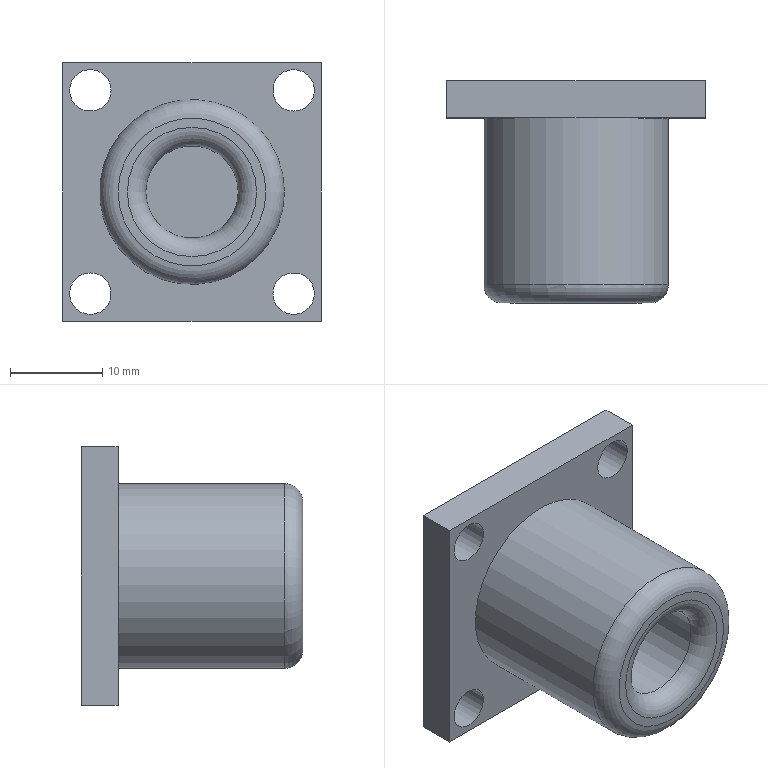Component | NX | INTERFACE_2 | 1 solid | 16 faces | box 28 x 24 x 28 mm | volume 7513 mm3 | plane 8 | cylinder 6 | torus 2 | commonest cylinder face diameters 4.5 x4 20 x1 10 x1
STEP:
#1=CARTESIAN_POINT('',(0.,0.,0.));
#2=DIRECTION('',(0.,0.,1.));
#3=DIRECTION('',(1.,0.,0.));
#4=AXIS2_PLACEMENT_3D('',#1,#2,#3);
#5=CARTESIAN_POINT('',(-14.,-309.,-187.));
#6=VERTEX_POINT('',#5);
#7=CARTESIAN_POINT('',(-14.,-309.,-215.));
#8=VERTEX_POINT('',#7);
#9=CARTESIAN_POINT('',(-14.,-309.,-187.));
#10=DIRECTION('',(0.,0.,-1.));
#11=VECTOR('',#10,1.);
#12=LINE('',#9,#11);
#13=CARTESIAN_POINT('',(-14.,-305.,-187.));
#14=DIRECTION('',(-1.,0.,0.));
#15=DIRECTION('',(0.,-1.,0.));
#16=AXIS2_PLACEMENT_3D('',#13,#14,#15);
#17=PLANE('',#16);
#18=CARTESIAN_POINT('',(4.,0.));
#19=DIRECTION('',(0.,-1.));
#20=VECTOR('',#19,1.);
#21=LINE('',#18,#20);
#22=(GEOMETRIC_REPRESENTATION_CONTEXT(2)PARAMETRIC_REPRESENTATION_CONTEXT()REPRESENTATION_CONTEXT('',''));
#23=DEFINITIONAL_REPRESENTATION('',(#21),#22);
#24=PCURVE('',#17,#23);
#25=CARTESIAN_POINT('',(-11.,-309.,-212.));
#26=DIRECTION('',(0.,-1.,0.));
#27=DIRECTION('',(1.,0.,0.));
#28=AXIS2_PLACEMENT_3D('',#25,#26,#27);
#29=PLANE('',#28);
#30=CARTESIAN_POINT('',(-3.,25.));
#31=DIRECTION('',(0.,-1.));
#32=VECTOR('',#31,1.);
#33=LINE('',#30,#32);
#34=(GEOMETRIC_REPRESENTATION_CONTEXT(2)PARAMETRIC_REPRESENTATION_CONTEXT()REPRESENTATION_CONTEXT('',''));
#35=DEFINITIONAL_REPRESENTATION('',(#33),#34);
#36=PCURVE('',#29,#35);
#37=SURFACE_CURVE('',#12,(#24,#36),.PCURVE_S1.);
#38=EDGE_CURVE('',#6,#8,#37,.T.);
#39=ORIENTED_EDGE('',*,*,#38,.F.);
#40=CARTESIAN_POINT('',(-14.,-305.,-187.));
#41=VERTEX_POINT('',#40);
#42=CARTESIAN_POINT('',(-14.,-305.,-187.));
#43=DIRECTION('',(0.,-1.,0.));
#44=VECTOR('',#43,1.);
#45=LINE('',#42,#44);
#46=CARTESIAN_POINT('',(0.,0.));
#47=DIRECTION('',(1.,0.));
#48=VECTOR('',#47,1.);
#49=LINE('',#46,#48);
#50=(GEOMETRIC_REPRESENTATION_CONTEXT(2)PARAMETRIC_REPRESENTATION_CONTEXT()REPRESENTATION_CONTEXT('',''));
#51=DEFINITIONAL_REPRESENTATION('',(#49),#50);
#52=PCURVE('',#17,#51);
#53=CARTESIAN_POINT('',(14.,-305.,-187.));
#54=DIRECTION('',(0.,0.,1.));
#55=DIRECTION('',(0.,-1.,0.));
#56=AXIS2_PLACEMENT_3D('',#53,#54,#55);
#57=PLANE('',#56);
#58=CARTESIAN_POINT('',(0.,-28.));
#59=DIRECTION('',(1.,0.));
#60=VECTOR('',#59,1.);
#61=LINE('',#58,#60);
#62=(GEOMETRIC_REPRESENTATION_CONTEXT(2)PARAMETRIC_REPRESENTATION_CONTEXT()REPRESENTATION_CONTEXT('',''));
#63=DEFINITIONAL_REPRESENTATION('',(#61),#62);
#64=PCURVE('',#57,#63);
#65=SURFACE_CURVE('',#45,(#52,#64),.PCURVE_S1.);
#66=EDGE_CURVE('',#41,#6,#65,.T.);
#67=ORIENTED_EDGE('',*,*,#66,.F.);
#68=CARTESIAN_POINT('',(-14.,-305.,-215.));
#69=VERTEX_POINT('',#68);
#70=CARTESIAN_POINT('',(-14.,-305.,-187.));
#71=DIRECTION('',(0.,0.,-1.));
#72=VECTOR('',#71,1.);
#73=LINE('',#70,#72);
#74=CARTESIAN_POINT('',(0.,0.));
#75=DIRECTION('',(0.,-1.));
#76=VECTOR('',#75,1.);
#77=LINE('',#74,#76);
#78=(GEOMETRIC_REPRESENTATION_CONTEXT(2)PARAMETRIC_REPRESENTATION_CONTEXT()REPRESENTATION_CONTEXT('',''));
#79=DEFINITIONAL_REPRESENTATION('',(#77),#78);
#80=PCURVE('',#17,#79);
#81=CARTESIAN_POINT('',(-11.,-305.,-212.));
#82=DIRECTION('',(0.,-1.,0.));
#83=DIRECTION('',(1.,0.,0.));
#84=AXIS2_PLACEMENT_3D('',#81,#82,#83);
#85=PLANE('',#84);
#86=CARTESIAN_POINT('',(-3.,25.));
#87=DIRECTION('',(0.,-1.));
#88=VECTOR('',#87,1.);
#89=LINE('',#86,#88);
#90=(GEOMETRIC_REPRESENTATION_CONTEXT(2)PARAMETRIC_REPRESENTATION_CONTEXT()REPRESENTATION_CONTEXT('',''));
#91=DEFINITIONAL_REPRESENTATION('',(#89),#90);
#92=PCURVE('',#85,#91);
#93=SURFACE_CURVE('',#73,(#80,#92),.PCURVE_S1.);
#94=EDGE_CURVE('',#41,#69,#93,.T.);
#95=ORIENTED_EDGE('',*,*,#94,.T.);
#96=CARTESIAN_POINT('',(-14.,-305.,-215.));
#97=DIRECTION('',(0.,-1.,0.));
#98=VECTOR('',#97,1.);
#99=LINE('',#96,#98);
#100=CARTESIAN_POINT('',(0.,-28.));
#101=DIRECTION('',(1.,0.));
#102=VECTOR('',#101,1.);
#103=LINE('',#100,#102);
#104=(GEOMETRIC_REPRESENTATION_CONTEXT(2)PARAMETRIC_REPRESENTATION_CONTEXT()REPRESENTATION_CONTEXT('',''));
#105=DEFINITIONAL_REPRESENTATION('',(#103),#104);
#106=PCURVE('',#17,#105);
#107=CARTESIAN_POINT('',(-14.,-305.,-215.));
#108=DIRECTION('',(0.,0.,-1.));
#109=DIRECTION('',(0.,1.,0.));
#110=AXIS2_PLACEMENT_3D('',#107,#108,#109);
#111=PLANE('',#110);
#112=CARTESIAN_POINT('',(0.,0.));
#113=DIRECTION('',(-1.,0.));
#114=VECTOR('',#113,1.);
#115=LINE('',#112,#114);
#116=(GEOMETRIC_REPRESENTATION_CONTEXT(2)PARAMETRIC_REPRESENTATION_CONTEXT()REPRESENTATION_CONTEXT('',''));
#117=DEFINITIONAL_REPRESENTATION('',(#115),#116);
#118=PCURVE('',#111,#117);
#119=SURFACE_CURVE('',#99,(#106,#118),.PCURVE_S1.);
#120=EDGE_CURVE('',#69,#8,#119,.T.);
#121=ORIENTED_EDGE('',*,*,#120,.T.);
#122=EDGE_LOOP('',(#39,#67,#95,#121));
#123=FACE_BOUND('',#122,.T.);
#124=ADVANCED_FACE('',(#123),#17,.T.);
#125=CARTESIAN_POINT('',(14.,-309.,-215.));
#126=VERTEX_POINT('',#125);
#127=CARTESIAN_POINT('',(-14.,-309.,-215.));
#128=DIRECTION('',(1.,0.,0.));
#129=VECTOR('',#128,1.);
#130=LINE('',#127,#129);
#131=CARTESIAN_POINT('',(-4.,0.));
#132=DIRECTION('',(0.,1.));
#133=VECTOR('',#132,1.);
#134=LINE('',#131,#133);
#135=(GEOMETRIC_REPRESENTATION_CONTEXT(2)PARAMETRIC_REPRESENTATION_CONTEXT()REPRESENTATION_CONTEXT('',''));
#136=DEFINITIONAL_REPRESENTATION('',(#134),#135);
#137=PCURVE('',#111,#136);
#138=CARTESIAN_POINT('',(-3.,-3.));
#139=DIRECTION('',(1.,0.));
#140=VECTOR('',#139,1.);
#141=LINE('',#138,#140);
#142=(GEOMETRIC_REPRESENTATION_CONTEXT(2)PARAMETRIC_REPRESENTATION_CONTEXT()REPRESENTATION_CONTEXT('',''));
#143=DEFINITIONAL_REPRESENTATION('',(#141),#142);
#144=PCURVE('',#29,#143);
#145=SURFACE_CURVE('',#130,(#137,#144),.PCURVE_S1.);
#146=EDGE_CURVE('',#8,#126,#145,.T.);
#147=ORIENTED_EDGE('',*,*,#146,.F.);
#148=ORIENTED_EDGE('',*,*,#120,.F.);
#149=CARTESIAN_POINT('',(14.,-305.,-215.));
#150=VERTEX_POINT('',#149);
#151=CARTESIAN_POINT('',(-14.,-305.,-215.));
#152=DIRECTION('',(1.,0.,0.));
#153=VECTOR('',#152,1.);
#154=LINE('',#151,#153);
#155=CARTESIAN_POINT('',(0.,0.));
#156=DIRECTION('',(0.,1.));
#157=VECTOR('',#156,1.);
#158=LINE('',#155,#157);
#159=(GEOMETRIC_REPRESENTATION_CONTEXT(2)PARAMETRIC_REPRESENTATION_CONTEXT()REPRESENTATION_CONTEXT('',''));
#160=DEFINITIONAL_REPRESENTATION('',(#158),#159);
#161=PCURVE('',#111,#160);
#162=CARTESIAN_POINT('',(-3.,-3.));
#163=DIRECTION('',(1.,0.));
#164=VECTOR('',#163,1.);
#165=LINE('',#162,#164);
#166=(GEOMETRIC_REPRESENTATION_CONTEXT(2)PARAMETRIC_REPRESENTATION_CONTEXT()REPRESENTATION_CONTEXT('',''));
#167=DEFINITIONAL_REPRESENTATION('',(#165),#166);
#168=PCURVE('',#85,#167);
#169=SURFACE_CURVE('',#154,(#161,#168),.PCURVE_S1.);
#170=EDGE_CURVE('',#69,#150,#169,.T.);
#171=ORIENTED_EDGE('',*,*,#170,.T.);
#172=CARTESIAN_POINT('',(14.,-305.,-215.));
#173=DIRECTION('',(0.,-1.,0.));
#174=VECTOR('',#173,1.);
#175=LINE('',#172,#174);
#176=CARTESIAN_POINT('',(0.,28.));
#177=DIRECTION('',(-1.,0.));
#178=VECTOR('',#177,1.);
#179=LINE('',#176,#178);
#180=(GEOMETRIC_REPRESENTATION_CONTEXT(2)PARAMETRIC_REPRESENTATION_CONTEXT()REPRESENTATION_CONTEXT('',''));
#181=DEFINITIONAL_REPRESENTATION('',(#179),#180);
#182=PCURVE('',#111,#181);
#183=CARTESIAN_POINT('',(14.,-305.,-215.));
#184=DIRECTION('',(1.,0.,0.));
#185=DIRECTION('',(0.,1.,0.));
#186=AXIS2_PLACEMENT_3D('',#183,#184,#185);
#187=PLANE('',#186);
#188=CARTESIAN_POINT('',(0.,0.));
#189=DIRECTION('',(-1.,0.));
#190=VECTOR('',#189,1.);
#191=LINE('',#188,#190);
#192=(GEOMETRIC_REPRESENTATION_CONTEXT(2)PARAMETRIC_REPRESENTATION_CONTEXT()REPRESENTATION_CONTEXT('',''));
#193=DEFINITIONAL_REPRESENTATION('',(#191),#192);
#194=PCURVE('',#187,#193);
#195=SURFACE_CURVE('',#175,(#182,#194),.PCURVE_S1.);
#196=EDGE_CURVE('',#150,#126,#195,.T.);
#197=ORIENTED_EDGE('',*,*,#196,.T.);
#198=EDGE_LOOP('',(#147,#148,#171,#197));
#199=FACE_BOUND('',#198,.T.);
#200=ADVANCED_FACE('',(#199),#111,.T.);
#201=CARTESIAN_POINT('',(14.,-309.,-187.));
#202=VERTEX_POINT('',#201);
#203=CARTESIAN_POINT('',(14.,-309.,-215.));
#204=DIRECTION('',(0.,0.,1.));
#205=VECTOR('',#204,1.);
#206=LINE('',#203,#205);
#207=CARTESIAN_POINT('',(-4.,0.));
#208=DIRECTION('',(0.,1.));
#209=VECTOR('',#208,1.);
#210=LINE('',#207,#209);
#211=(GEOMETRIC_REPRESENTATION_CONTEXT(2)PARAMETRIC_REPRESENTATION_CONTEXT()REPRESENTATION_CONTEXT('',''));
#212=DEFINITIONAL_REPRESENTATION('',(#210),#211);
#213=PCURVE('',#187,#212);
#214=CARTESIAN_POINT('',(25.,-3.));
#215=DIRECTION('',(0.,1.));
#216=VECTOR('',#215,1.);
#217=LINE('',#214,#216);
#218=(GEOMETRIC_REPRESENTATION_CONTEXT(2)PARAMETRIC_REPRESENTATION_CONTEXT()REPRESENTATION_CONTEXT('',''));
#219=DEFINITIONAL_REPRESENTATION('',(#217),#218);
#220=PCURVE('',#29,#219);
#221=SURFACE_CURVE('',#206,(#213,#220),.PCURVE_S1.);
#222=EDGE_CURVE('',#126,#202,#221,.T.);
#223=ORIENTED_EDGE('',*,*,#222,.F.);
#224=ORIENTED_EDGE('',*,*,#196,.F.);
#225=CARTESIAN_POINT('',(14.,-305.,-187.));
#226=VERTEX_POINT('',#225);
#227=CARTESIAN_POINT('',(14.,-305.,-215.));
#228=DIRECTION('',(0.,0.,1.));
#229=VECTOR('',#228,1.);
#230=LINE('',#227,#229);
#231=CARTESIAN_POINT('',(0.,0.));
#232=DIRECTION('',(0.,1.));
#233=VECTOR('',#232,1.);
#234=LINE('',#231,#233);
#235=(GEOMETRIC_REPRESENTATION_CONTEXT(2)PARAMETRIC_REPRESENTATION_CONTEXT()REPRESENTATION_CONTEXT('',''));
#236=DEFINITIONAL_REPRESENTATION('',(#234),#235);
#237=PCURVE('',#187,#236);
#238=CARTESIAN_POINT('',(25.,-3.));
#239=DIRECTION('',(0.,1.));
#240=VECTOR('',#239,1.);
#241=LINE('',#238,#240);
#242=(GEOMETRIC_REPRESENTATION_CONTEXT(2)PARAMETRIC_REPRESENTATION_CONTEXT()REPRESENTATION_CONTEXT('',''));
#243=DEFINITIONAL_REPRESENTATION('',(#241),#242);
#244=PCURVE('',#85,#243);
#245=SURFACE_CURVE('',#230,(#237,#244),.PCURVE_S1.);
#246=EDGE_CURVE('',#150,#226,#245,.T.);
#247=ORIENTED_EDGE('',*,*,#246,.T.);
#248=CARTESIAN_POINT('',(14.,-305.,-187.));
#249=DIRECTION('',(0.,-1.,0.));
#250=VECTOR('',#249,1.);
#251=LINE('',#248,#250);
#252=CARTESIAN_POINT('',(0.,28.));
#253=DIRECTION('',(-1.,0.));
#254=VECTOR('',#253,1.);
#255=LINE('',#252,#254);
#256=(GEOMETRIC_REPRESENTATION_CONTEXT(2)PARAMETRIC_REPRESENTATION_CONTEXT()REPRESENTATION_CONTEXT('',''));
#257=DEFINITIONAL_REPRESENTATION('',(#255),#256);
#258=PCURVE('',#187,#257);
#259=CARTESIAN_POINT('',(0.,0.));
#260=DIRECTION('',(1.,0.));
#261=VECTOR('',#260,1.);
#262=LINE('',#259,#261);
#263=(GEOMETRIC_REPRESENTATION_CONTEXT(2)PARAMETRIC_REPRESENTATION_CONTEXT()REPRESENTATION_CONTEXT('',''));
#264=DEFINITIONAL_REPRESENTATION('',(#262),#263);
#265=PCURVE('',#57,#264);
#266=SURFACE_CURVE('',#251,(#258,#265),.PCURVE_S1.);
#267=EDGE_CURVE('',#226,#202,#266,.T.);
#268=ORIENTED_EDGE('',*,*,#267,.T.);
#269=EDGE_LOOP('',(#223,#224,#247,#268));
#270=FACE_BOUND('',#269,.T.);
#271=ADVANCED_FACE('',(#270),#187,.T.);
#272=CARTESIAN_POINT('',(8.75,-305.,-212.));
#273=VERTEX_POINT('',#272);
#274=CARTESIAN_POINT('',(11.,-305.,-212.));
#275=DIRECTION('',(0.,-1.,0.));
#276=DIRECTION('',(-1.,0.,0.));
#277=AXIS2_PLACEMENT_3D('',#274,#275,#276);
#278=CIRCLE('',#277,2.25);
#279=CARTESIAN_POINT('',(11.,-305.,-212.));
#280=DIRECTION('',(0.,-1.,0.));
#281=DIRECTION('',(1.,0.,0.));
#282=AXIS2_PLACEMENT_3D('',#279,#280,#281);
#283=CYLINDRICAL_SURFACE('',#282,2.25);
#284=CARTESIAN_POINT('',(3.142,0.));
#285=DIRECTION('',(1.,0.));
#286=VECTOR('',#285,1.);
#287=LINE('',#284,#286);
#288=(GEOMETRIC_REPRESENTATION_CONTEXT(2)PARAMETRIC_REPRESENTATION_CONTEXT()REPRESENTATION_CONTEXT('',''));
#289=DEFINITIONAL_REPRESENTATION('',(#287),#288);
#290=PCURVE('',#283,#289);
#291=CARTESIAN_POINT('',(22.,0.));
#292=DIRECTION('',(-1.,0.));
#293=AXIS2_PLACEMENT_2D('',#291,#292);
#294=CIRCLE('',#293,2.25);
#295=(GEOMETRIC_REPRESENTATION_CONTEXT(2)PARAMETRIC_REPRESENTATION_CONTEXT()REPRESENTATION_CONTEXT('',''));
#296=DEFINITIONAL_REPRESENTATION('',(#294),#295);
#297=PCURVE('',#85,#296);
#298=SURFACE_CURVE('',#278,(#290,#297),.PCURVE_S1.);
#299=EDGE_CURVE('',#273,#273,#298,.T.);
#300=ORIENTED_EDGE('',*,*,#299,.T.);
#301=CARTESIAN_POINT('',(8.75,-309.,-212.));
#302=VERTEX_POINT('',#301);
#303=CARTESIAN_POINT('',(8.75,-305.,-212.));
#304=CARTESIAN_POINT('',(8.75,-309.,-212.));
#305=B_SPLINE_CURVE_WITH_KNOTS('',1,(#303,#304),.UNSPECIFIED.,.F.,.F.,(2,2),(0.,4.),.PIECEWISE_BEZIER_KNOTS.);
#306=CARTESIAN_POINT('',(9.425,0.));
#307=DIRECTION('',(0.,1.));
#308=VECTOR('',#307,1.);
#309=LINE('',#306,#308);
#310=(GEOMETRIC_REPRESENTATION_CONTEXT(2)PARAMETRIC_REPRESENTATION_CONTEXT()REPRESENTATION_CONTEXT('',''));
#311=DEFINITIONAL_REPRESENTATION('',(#309),#310);
#312=PCURVE('',#283,#311);
#313=CARTESIAN_POINT('',(3.142,0.));
#314=DIRECTION('',(0.,1.));
#315=VECTOR('',#314,1.);
#316=LINE('',#313,#315);
#317=(GEOMETRIC_REPRESENTATION_CONTEXT(2)PARAMETRIC_REPRESENTATION_CONTEXT()REPRESENTATION_CONTEXT('',''));
#318=DEFINITIONAL_REPRESENTATION('',(#316),#317);
#319=PCURVE('',#283,#318);
#320=SEAM_CURVE('',#305,(#312,#319),.PCURVE_S1.);
#321=EDGE_CURVE('',#273,#302,#320,.T.);
#322=ORIENTED_EDGE('',*,*,#321,.T.);
#323=CARTESIAN_POINT('',(11.,-309.,-212.));
#324=DIRECTION('',(0.,-1.,0.));
#325=DIRECTION('',(-1.,0.,0.));
#326=AXIS2_PLACEMENT_3D('',#323,#324,#325);
#327=CIRCLE('',#326,2.25);
#328=CARTESIAN_POINT('',(3.142,4.));
#329=DIRECTION('',(1.,0.));
#330=VECTOR('',#329,1.);
#331=LINE('',#328,#330);
#332=(GEOMETRIC_REPRESENTATION_CONTEXT(2)PARAMETRIC_REPRESENTATION_CONTEXT()REPRESENTATION_CONTEXT('',''));
#333=DEFINITIONAL_REPRESENTATION('',(#331),#332);
#334=PCURVE('',#283,#333);
#335=CARTESIAN_POINT('',(22.,0.));
#336=DIRECTION('',(-1.,0.));
#337=AXIS2_PLACEMENT_2D('',#335,#336);
#338=CIRCLE('',#337,2.25);
#339=(GEOMETRIC_REPRESENTATION_CONTEXT(2)PARAMETRIC_REPRESENTATION_CONTEXT()REPRESENTATION_CONTEXT('',''));
#340=DEFINITIONAL_REPRESENTATION('',(#338),#339);
#341=PCURVE('',#29,#340);
#342=SURFACE_CURVE('',#327,(#334,#341),.PCURVE_S1.);
#343=EDGE_CURVE('',#302,#302,#342,.T.);
#344=ORIENTED_EDGE('',*,*,#343,.F.);
#345=ORIENTED_EDGE('',*,*,#321,.F.);
#346=EDGE_LOOP('',(#300,#322,#344,#345));
#347=FACE_BOUND('',#346,.F.);
#348=ADVANCED_FACE('',(#347),#283,.F.);
#349=CARTESIAN_POINT('',(-8.75,-305.,-190.));
#350=VERTEX_POINT('',#349);
#351=CARTESIAN_POINT('',(-11.,-305.,-190.));
#352=DIRECTION('',(0.,-1.,0.));
#353=DIRECTION('',(1.,0.,0.));
#354=AXIS2_PLACEMENT_3D('',#351,#352,#353);
#355=CIRCLE('',#354,2.25);
#356=CARTESIAN_POINT('',(-11.,-305.,-190.));
#357=DIRECTION('',(0.,-1.,0.));
#358=DIRECTION('',(1.,0.,0.));
#359=AXIS2_PLACEMENT_3D('',#356,#357,#358);
#360=CYLINDRICAL_SURFACE('',#359,2.25);
#361=CARTESIAN_POINT('',(0.,0.));
#362=DIRECTION('',(1.,0.));
#363=VECTOR('',#362,1.);
#364=LINE('',#361,#363);
#365=(GEOMETRIC_REPRESENTATION_CONTEXT(2)PARAMETRIC_REPRESENTATION_CONTEXT()REPRESENTATION_CONTEXT('',''));
#366=DEFINITIONAL_REPRESENTATION('',(#364),#365);
#367=PCURVE('',#360,#366);
#368=CARTESIAN_POINT('',(0.,22.));
#369=DIRECTION('',(1.,0.));
#370=AXIS2_PLACEMENT_2D('',#368,#369);
#371=CIRCLE('',#370,2.25);
#372=(GEOMETRIC_REPRESENTATION_CONTEXT(2)PARAMETRIC_REPRESENTATION_CONTEXT()REPRESENTATION_CONTEXT('',''));
#373=DEFINITIONAL_REPRESENTATION('',(#371),#372);
#374=PCURVE('',#85,#373);
#375=SURFACE_CURVE('',#355,(#367,#374),.PCURVE_S1.);
#376=EDGE_CURVE('',#350,#350,#375,.T.);
#377=ORIENTED_EDGE('',*,*,#376,.T.);
#378=CARTESIAN_POINT('',(-8.75,-309.,-190.));
#379=VERTEX_POINT('',#378);
#380=CARTESIAN_POINT('',(-8.75,-305.,-190.));
#381=CARTESIAN_POINT('',(-8.75,-309.,-190.));
#382=B_SPLINE_CURVE_WITH_KNOTS('',1,(#380,#381),.UNSPECIFIED.,.F.,.F.,(2,2),(0.,4.),.PIECEWISE_BEZIER_KNOTS.);
#383=CARTESIAN_POINT('',(6.283,0.));
#384=DIRECTION('',(0.,1.));
#385=VECTOR('',#384,1.);
#386=LINE('',#383,#385);
#387=(GEOMETRIC_REPRESENTATION_CONTEXT(2)PARAMETRIC_REPRESENTATION_CONTEXT()REPRESENTATION_CONTEXT('',''));
#388=DEFINITIONAL_REPRESENTATION('',(#386),#387);
#389=PCURVE('',#360,#388);
#390=CARTESIAN_POINT('',(0.,0.));
#391=DIRECTION('',(0.,1.));
#392=VECTOR('',#391,1.);
#393=LINE('',#390,#392);
#394=(GEOMETRIC_REPRESENTATION_CONTEXT(2)PARAMETRIC_REPRESENTATION_CONTEXT()REPRESENTATION_CONTEXT('',''));
#395=DEFINITIONAL_REPRESENTATION('',(#393),#394);
#396=PCURVE('',#360,#395);
#397=SEAM_CURVE('',#382,(#389,#396),.PCURVE_S1.);
#398=EDGE_CURVE('',#350,#379,#397,.T.);
#399=ORIENTED_EDGE('',*,*,#398,.T.);
#400=CARTESIAN_POINT('',(-11.,-309.,-190.));
#401=DIRECTION('',(0.,-1.,0.));
#402=DIRECTION('',(1.,0.,0.));
#403=AXIS2_PLACEMENT_3D('',#400,#401,#402);
#404=CIRCLE('',#403,2.25);
#405=CARTESIAN_POINT('',(0.,4.));
#406=DIRECTION('',(1.,0.));
#407=VECTOR('',#406,1.);
#408=LINE('',#405,#407);
#409=(GEOMETRIC_REPRESENTATION_CONTEXT(2)PARAMETRIC_REPRESENTATION_CONTEXT()REPRESENTATION_CONTEXT('',''));
#410=DEFINITIONAL_REPRESENTATION('',(#408),#409);
#411=PCURVE('',#360,#410);
#412=CARTESIAN_POINT('',(0.,22.));
#413=DIRECTION('',(1.,0.));
#414=AXIS2_PLACEMENT_2D('',#412,#413);
#415=CIRCLE('',#414,2.25);
#416=(GEOMETRIC_REPRESENTATION_CONTEXT(2)PARAMETRIC_REPRESENTATION_CONTEXT()REPRESENTATION_CONTEXT('',''));
#417=DEFINITIONAL_REPRESENTATION('',(#415),#416);
#418=PCURVE('',#29,#417);
#419=SURFACE_CURVE('',#404,(#411,#418),.PCURVE_S1.);
#420=EDGE_CURVE('',#379,#379,#419,.T.);
#421=ORIENTED_EDGE('',*,*,#420,.F.);
#422=ORIENTED_EDGE('',*,*,#398,.F.);
#423=EDGE_LOOP('',(#377,#399,#421,#422));
#424=FACE_BOUND('',#423,.F.);
#425=ADVANCED_FACE('',(#424),#360,.F.);
#426=CARTESIAN_POINT('',(-11.,-305.,-209.75));
#427=VERTEX_POINT('',#426);
#428=CARTESIAN_POINT('',(-11.,-305.,-212.));
#429=DIRECTION('',(0.,-1.,0.));
#430=DIRECTION('',(0.,0.,1.));
#431=AXIS2_PLACEMENT_3D('',#428,#429,#430);
#432=CIRCLE('',#431,2.25);
#433=CARTESIAN_POINT('',(-11.,-305.,-212.));
#434=DIRECTION('',(0.,-1.,0.));
#435=DIRECTION('',(1.,0.,0.));
#436=AXIS2_PLACEMENT_3D('',#433,#434,#435);
#437=CYLINDRICAL_SURFACE('',#436,2.25);
#438=CARTESIAN_POINT('',(1.571,0.));
#439=DIRECTION('',(1.,0.));
#440=VECTOR('',#439,1.);
#441=LINE('',#438,#440);
#442=(GEOMETRIC_REPRESENTATION_CONTEXT(2)PARAMETRIC_REPRESENTATION_CONTEXT()REPRESENTATION_CONTEXT('',''));
#443=DEFINITIONAL_REPRESENTATION('',(#441),#442);
#444=PCURVE('',#437,#443);
#445=CARTESIAN_POINT('',(0.,0.));
#446=DIRECTION('',(0.,1.));
#447=AXIS2_PLACEMENT_2D('',#445,#446);
#448=CIRCLE('',#447,2.25);
#449=(GEOMETRIC_REPRESENTATION_CONTEXT(2)PARAMETRIC_REPRESENTATION_CONTEXT()REPRESENTATION_CONTEXT('',''));
#450=DEFINITIONAL_REPRESENTATION('',(#448),#449);
#451=PCURVE('',#85,#450);
#452=SURFACE_CURVE('',#432,(#444,#451),.PCURVE_S1.);
#453=EDGE_CURVE('',#427,#427,#452,.T.);
#454=ORIENTED_EDGE('',*,*,#453,.T.);
#455=CARTESIAN_POINT('',(-11.,-309.,-209.75));
#456=VERTEX_POINT('',#455);
#457=CARTESIAN_POINT('',(-11.,-305.,-209.75));
#458=CARTESIAN_POINT('',(-11.,-309.,-209.75));
#459=B_SPLINE_CURVE_WITH_KNOTS('',1,(#457,#458),.UNSPECIFIED.,.F.,.F.,(2,2),(0.,4.),.PIECEWISE_BEZIER_KNOTS.);
#460=CARTESIAN_POINT('',(7.854,0.));
#461=DIRECTION('',(0.,1.));
#462=VECTOR('',#461,1.);
#463=LINE('',#460,#462);
#464=(GEOMETRIC_REPRESENTATION_CONTEXT(2)PARAMETRIC_REPRESENTATION_CONTEXT()REPRESENTATION_CONTEXT('',''));
#465=DEFINITIONAL_REPRESENTATION('',(#463),#464);
#466=PCURVE('',#437,#465);
#467=CARTESIAN_POINT('',(1.571,0.));
#468=DIRECTION('',(0.,1.));
#469=VECTOR('',#468,1.);
#470=LINE('',#467,#469);
#471=(GEOMETRIC_REPRESENTATION_CONTEXT(2)PARAMETRIC_REPRESENTATION_CONTEXT()REPRESENTATION_CONTEXT('',''));
#472=DEFINITIONAL_REPRESENTATION('',(#470),#471);
#473=PCURVE('',#437,#472);
#474=SEAM_CURVE('',#459,(#466,#473),.PCURVE_S1.);
#475=EDGE_CURVE('',#427,#456,#474,.T.);
#476=ORIENTED_EDGE('',*,*,#475,.T.);
#477=CARTESIAN_POINT('',(-11.,-309.,-212.));
#478=DIRECTION('',(0.,-1.,0.));
#479=DIRECTION('',(0.,0.,1.));
#480=AXIS2_PLACEMENT_3D('',#477,#478,#479);
#481=CIRCLE('',#480,2.25);
#482=CARTESIAN_POINT('',(1.571,4.));
#483=DIRECTION('',(1.,0.));
#484=VECTOR('',#483,1.);
#485=LINE('',#482,#484);
#486=(GEOMETRIC_REPRESENTATION_CONTEXT(2)PARAMETRIC_REPRESENTATION_CONTEXT()REPRESENTATION_CONTEXT('',''));
#487=DEFINITIONAL_REPRESENTATION('',(#485),#486);
#488=PCURVE('',#437,#487);
#489=CARTESIAN_POINT('',(0.,0.));
#490=DIRECTION('',(0.,1.));
#491=AXIS2_PLACEMENT_2D('',#489,#490);
#492=CIRCLE('',#491,2.25);
#493=(GEOMETRIC_REPRESENTATION_CONTEXT(2)PARAMETRIC_REPRESENTATION_CONTEXT()REPRESENTATION_CONTEXT('',''));
#494=DEFINITIONAL_REPRESENTATION('',(#492),#493);
#495=PCURVE('',#29,#494);
#496=SURFACE_CURVE('',#481,(#488,#495),.PCURVE_S1.);
#497=EDGE_CURVE('',#456,#456,#496,.T.);
#498=ORIENTED_EDGE('',*,*,#497,.F.);
#499=ORIENTED_EDGE('',*,*,#475,.F.);
#500=EDGE_LOOP('',(#454,#476,#498,#499));
#501=FACE_BOUND('',#500,.F.);
#502=ADVANCED_FACE('',(#501),#437,.F.);
#503=CARTESIAN_POINT('',(14.,-309.,-187.));
#504=DIRECTION('',(-1.,0.,0.));
#505=VECTOR('',#504,1.);
#506=LINE('',#503,#505);
#507=CARTESIAN_POINT('',(4.,0.));
#508=DIRECTION('',(0.,-1.));
#509=VECTOR('',#508,1.);
#510=LINE('',#507,#509);
#511=(GEOMETRIC_REPRESENTATION_CONTEXT(2)PARAMETRIC_REPRESENTATION_CONTEXT()REPRESENTATION_CONTEXT('',''));
#512=DEFINITIONAL_REPRESENTATION('',(#510),#511);
#513=PCURVE('',#57,#512);
#514=CARTESIAN_POINT('',(25.,25.));
#515=DIRECTION('',(-1.,0.));
#516=VECTOR('',#515,1.);
#517=LINE('',#514,#516);
#518=(GEOMETRIC_REPRESENTATION_CONTEXT(2)PARAMETRIC_REPRESENTATION_CONTEXT()REPRESENTATION_CONTEXT('',''));
#519=DEFINITIONAL_REPRESENTATION('',(#517),#518);
#520=PCURVE('',#29,#519);
#521=SURFACE_CURVE('',#506,(#513,#520),.PCURVE_S1.);
#522=EDGE_CURVE('',#202,#6,#521,.T.);
#523=ORIENTED_EDGE('',*,*,#522,.F.);
#524=ORIENTED_EDGE('',*,*,#267,.F.);
#525=CARTESIAN_POINT('',(14.,-305.,-187.));
#526=DIRECTION('',(-1.,0.,0.));
#527=VECTOR('',#526,1.);
#528=LINE('',#525,#527);
#529=CARTESIAN_POINT('',(0.,0.));
#530=DIRECTION('',(0.,-1.));
#531=VECTOR('',#530,1.);
#532=LINE('',#529,#531);
#533=(GEOMETRIC_REPRESENTATION_CONTEXT(2)PARAMETRIC_REPRESENTATION_CONTEXT()REPRESENTATION_CONTEXT('',''));
#534=DEFINITIONAL_REPRESENTATION('',(#532),#533);
#535=PCURVE('',#57,#534);
#536=CARTESIAN_POINT('',(25.,25.));
#537=DIRECTION('',(-1.,0.));
#538=VECTOR('',#537,1.);
#539=LINE('',#536,#538);
#540=(GEOMETRIC_REPRESENTATION_CONTEXT(2)PARAMETRIC_REPRESENTATION_CONTEXT()REPRESENTATION_CONTEXT('',''));
#541=DEFINITIONAL_REPRESENTATION('',(#539),#540);
#542=PCURVE('',#85,#541);
#543=SURFACE_CURVE('',#528,(#535,#542),.PCURVE_S1.);
#544=EDGE_CURVE('',#226,#41,#543,.T.);
#545=ORIENTED_EDGE('',*,*,#544,.T.);
#546=ORIENTED_EDGE('',*,*,#66,.T.);
#547=EDGE_LOOP('',(#523,#524,#545,#546));
#548=FACE_BOUND('',#547,.T.);
#549=ADVANCED_FACE('',(#548),#57,.T.);
#550=CARTESIAN_POINT('',(11.,-305.,-192.25));
#551=VERTEX_POINT('',#550);
#552=CARTESIAN_POINT('',(11.,-305.,-190.));
#553=DIRECTION('',(0.,-1.,0.));
#554=DIRECTION('',(0.,0.,-1.));
#555=AXIS2_PLACEMENT_3D('',#552,#553,#554);
#556=CIRCLE('',#555,2.25);
#557=CARTESIAN_POINT('',(11.,-305.,-190.));
#558=DIRECTION('',(0.,-1.,0.));
#559=DIRECTION('',(1.,0.,0.));
#560=AXIS2_PLACEMENT_3D('',#557,#558,#559);
#561=CYLINDRICAL_SURFACE('',#560,2.25);
#562=CARTESIAN_POINT('',(4.712,0.));
#563=DIRECTION('',(1.,0.));
#564=VECTOR('',#563,1.);
#565=LINE('',#562,#564);
#566=(GEOMETRIC_REPRESENTATION_CONTEXT(2)PARAMETRIC_REPRESENTATION_CONTEXT()REPRESENTATION_CONTEXT('',''));
#567=DEFINITIONAL_REPRESENTATION('',(#565),#566);
#568=PCURVE('',#561,#567);
#569=CARTESIAN_POINT('',(22.,22.));
#570=DIRECTION('',(0.,-1.));
#571=AXIS2_PLACEMENT_2D('',#569,#570);
#572=CIRCLE('',#571,2.25);
#573=(GEOMETRIC_REPRESENTATION_CONTEXT(2)PARAMETRIC_REPRESENTATION_CONTEXT()REPRESENTATION_CONTEXT('',''));
#574=DEFINITIONAL_REPRESENTATION('',(#572),#573);
#575=PCURVE('',#85,#574);
#576=SURFACE_CURVE('',#556,(#568,#575),.PCURVE_S1.);
#577=EDGE_CURVE('',#551,#551,#576,.T.);
#578=ORIENTED_EDGE('',*,*,#577,.T.);
#579=CARTESIAN_POINT('',(11.,-309.,-192.25));
#580=VERTEX_POINT('',#579);
#581=CARTESIAN_POINT('',(11.,-305.,-192.25));
#582=CARTESIAN_POINT('',(11.,-309.,-192.25));
#583=B_SPLINE_CURVE_WITH_KNOTS('',1,(#581,#582),.UNSPECIFIED.,.F.,.F.,(2,2),(0.,4.),.PIECEWISE_BEZIER_KNOTS.);
#584=CARTESIAN_POINT('',(10.996,0.));
#585=DIRECTION('',(0.,1.));
#586=VECTOR('',#585,1.);
#587=LINE('',#584,#586);
#588=(GEOMETRIC_REPRESENTATION_CONTEXT(2)PARAMETRIC_REPRESENTATION_CONTEXT()REPRESENTATION_CONTEXT('',''));
#589=DEFINITIONAL_REPRESENTATION('',(#587),#588);
#590=PCURVE('',#561,#589);
#591=CARTESIAN_POINT('',(4.712,0.));
#592=DIRECTION('',(0.,1.));
#593=VECTOR('',#592,1.);
#594=LINE('',#591,#593);
#595=(GEOMETRIC_REPRESENTATION_CONTEXT(2)PARAMETRIC_REPRESENTATION_CONTEXT()REPRESENTATION_CONTEXT('',''));
#596=DEFINITIONAL_REPRESENTATION('',(#594),#595);
#597=PCURVE('',#561,#596);
#598=SEAM_CURVE('',#583,(#590,#597),.PCURVE_S1.);
#599=EDGE_CURVE('',#551,#580,#598,.T.);
#600=ORIENTED_EDGE('',*,*,#599,.T.);
#601=CARTESIAN_POINT('',(11.,-309.,-190.));
#602=DIRECTION('',(0.,-1.,0.));
#603=DIRECTION('',(0.,0.,-1.));
#604=AXIS2_PLACEMENT_3D('',#601,#602,#603);
#605=CIRCLE('',#604,2.25);
#606=CARTESIAN_POINT('',(4.712,4.));
#607=DIRECTION('',(1.,0.));
#608=VECTOR('',#607,1.);
#609=LINE('',#606,#608);
#610=(GEOMETRIC_REPRESENTATION_CONTEXT(2)PARAMETRIC_REPRESENTATION_CONTEXT()REPRESENTATION_CONTEXT('',''));
#611=DEFINITIONAL_REPRESENTATION('',(#609),#610);
#612=PCURVE('',#561,#611);
#613=CARTESIAN_POINT('',(22.,22.));
#614=DIRECTION('',(0.,-1.));
#615=AXIS2_PLACEMENT_2D('',#613,#614);
#616=CIRCLE('',#615,2.25);
#617=(GEOMETRIC_REPRESENTATION_CONTEXT(2)PARAMETRIC_REPRESENTATION_CONTEXT()REPRESENTATION_CONTEXT('',''));
#618=DEFINITIONAL_REPRESENTATION('',(#616),#617);
#619=PCURVE('',#29,#618);
#620=SURFACE_CURVE('',#605,(#612,#619),.PCURVE_S1.);
#621=EDGE_CURVE('',#580,#580,#620,.T.);
#622=ORIENTED_EDGE('',*,*,#621,.F.);
#623=ORIENTED_EDGE('',*,*,#599,.F.);
#624=EDGE_LOOP('',(#578,#600,#622,#623));
#625=FACE_BOUND('',#624,.F.);
#626=ADVANCED_FACE('',(#625),#561,.F.);
#627=ORIENTED_EDGE('',*,*,#94,.F.);
#628=ORIENTED_EDGE('',*,*,#544,.F.);
#629=ORIENTED_EDGE('',*,*,#246,.F.);
#630=ORIENTED_EDGE('',*,*,#170,.F.);
#631=EDGE_LOOP('',(#627,#628,#629,#630));
#632=FACE_BOUND('',#631,.T.);
#633=ORIENTED_EDGE('',*,*,#453,.T.);
#634=EDGE_LOOP('',(#633));
#635=FACE_BOUND('',#634,.T.);
#636=ORIENTED_EDGE('',*,*,#376,.T.);
#637=EDGE_LOOP('',(#636));
#638=FACE_BOUND('',#637,.T.);
#639=ORIENTED_EDGE('',*,*,#299,.T.);
#640=EDGE_LOOP('',(#639));
#641=FACE_BOUND('',#640,.T.);
#642=ORIENTED_EDGE('',*,*,#577,.T.);
#643=EDGE_LOOP('',(#642));
#644=FACE_BOUND('',#643,.T.);
#645=ADVANCED_FACE('',(#632,#635,#638,#641,#644),#85,.F.);
#646=CARTESIAN_POINT('',(10.,-309.,-201.));
#647=VERTEX_POINT('',#646);
#648=CARTESIAN_POINT('',(0.,-309.,-201.));
#649=DIRECTION('',(0.,-1.,0.));
#650=DIRECTION('',(1.,0.,0.));
#651=AXIS2_PLACEMENT_3D('',#648,#649,#650);
#652=CIRCLE('',#651,10.);
#653=CARTESIAN_POINT('',(11.,11.));
#654=DIRECTION('',(1.,0.));
#655=AXIS2_PLACEMENT_2D('',#653,#654);
#656=CIRCLE('',#655,10.);
#657=(GEOMETRIC_REPRESENTATION_CONTEXT(2)PARAMETRIC_REPRESENTATION_CONTEXT()REPRESENTATION_CONTEXT('',''));
#658=DEFINITIONAL_REPRESENTATION('',(#656),#657);
#659=PCURVE('',#29,#658);
#660=CARTESIAN_POINT('',(0.,-329.,-201.));
#661=DIRECTION('',(0.,1.,0.));
#662=DIRECTION('',(-1.,0.,0.));
#663=AXIS2_PLACEMENT_3D('',#660,#661,#662);
#664=CYLINDRICAL_SURFACE('',#663,10.);
#665=CARTESIAN_POINT('',(9.425,20.));
#666=DIRECTION('',(-1.,0.));
#667=VECTOR('',#666,1.);
#668=LINE('',#665,#667);
#669=(GEOMETRIC_REPRESENTATION_CONTEXT(2)PARAMETRIC_REPRESENTATION_CONTEXT()REPRESENTATION_CONTEXT('',''));
#670=DEFINITIONAL_REPRESENTATION('',(#668),#669);
#671=PCURVE('',#664,#670);
#672=SURFACE_CURVE('',#652,(#659,#671),.PCURVE_S1.);
#673=EDGE_CURVE('',#647,#647,#672,.T.);
#674=ORIENTED_EDGE('',*,*,#673,.F.);
#675=EDGE_LOOP('',(#674));
#676=FACE_BOUND('',#675,.T.);
#677=ORIENTED_EDGE('',*,*,#38,.T.);
#678=ORIENTED_EDGE('',*,*,#146,.T.);
#679=ORIENTED_EDGE('',*,*,#222,.T.);
#680=ORIENTED_EDGE('',*,*,#522,.T.);
#681=EDGE_LOOP('',(#677,#678,#679,#680));
#682=FACE_BOUND('',#681,.T.);
#683=ORIENTED_EDGE('',*,*,#497,.F.);
#684=EDGE_LOOP('',(#683));
#685=FACE_BOUND('',#684,.T.);
#686=ORIENTED_EDGE('',*,*,#420,.F.);
#687=EDGE_LOOP('',(#686));
#688=FACE_BOUND('',#687,.T.);
#689=ORIENTED_EDGE('',*,*,#343,.F.);
#690=EDGE_LOOP('',(#689));
#691=FACE_BOUND('',#690,.T.);
#692=ORIENTED_EDGE('',*,*,#621,.F.);
#693=EDGE_LOOP('',(#692));
#694=FACE_BOUND('',#693,.T.);
#695=ADVANCED_FACE('',(#676,#682,#685,#688,#691,#694),#29,.T.);
#696=CARTESIAN_POINT('',(10.,-327.,-201.));
#697=VERTEX_POINT('',#696);
#698=CARTESIAN_POINT('',(0.,-327.,-201.));
#699=DIRECTION('',(0.,1.,0.));
#700=DIRECTION('',(1.,0.,0.));
#701=AXIS2_PLACEMENT_3D('',#698,#699,#700);
#702=CIRCLE('',#701,10.);
#703=CARTESIAN_POINT('',(3.142,2.));
#704=DIRECTION('',(1.,0.));
#705=VECTOR('',#704,1.);
#706=LINE('',#703,#705);
#707=(GEOMETRIC_REPRESENTATION_CONTEXT(2)PARAMETRIC_REPRESENTATION_CONTEXT()REPRESENTATION_CONTEXT('',''));
#708=DEFINITIONAL_REPRESENTATION('',(#706),#707);
#709=PCURVE('',#664,#708);
#710=CARTESIAN_POINT('',(0.,-327.,-201.));
#711=DIRECTION('',(0.,-1.,0.));
#712=DIRECTION('',(1.,0.,0.));
#713=AXIS2_PLACEMENT_3D('',#710,#711,#712);
#714=TOROIDAL_SURFACE('',#713,8.,2.);
#715=CARTESIAN_POINT('',(6.283,6.283));
#716=DIRECTION('',(-1.,0.));
#717=VECTOR('',#716,1.);
#718=LINE('',#715,#717);
#719=(GEOMETRIC_REPRESENTATION_CONTEXT(2)PARAMETRIC_REPRESENTATION_CONTEXT()REPRESENTATION_CONTEXT('',''));
#720=DEFINITIONAL_REPRESENTATION('',(#718),#719);
#721=PCURVE('',#714,#720);
#722=SURFACE_CURVE('',#702,(#709,#721),.PCURVE_S1.);
#723=EDGE_CURVE('',#697,#697,#722,.T.);
#724=ORIENTED_EDGE('',*,*,#723,.T.);
#725=CARTESIAN_POINT('',(10.,-327.,-201.));
#726=CARTESIAN_POINT('',(10.,-309.,-201.));
#727=B_SPLINE_CURVE_WITH_KNOTS('',1,(#725,#726),.UNSPECIFIED.,.F.,.F.,(2,2),(2.,20.),.PIECEWISE_BEZIER_KNOTS.);
#728=CARTESIAN_POINT('',(9.425,0.));
#729=DIRECTION('',(0.,1.));
#730=VECTOR('',#729,1.);
#731=LINE('',#728,#730);
#732=(GEOMETRIC_REPRESENTATION_CONTEXT(2)PARAMETRIC_REPRESENTATION_CONTEXT()REPRESENTATION_CONTEXT('',''));
#733=DEFINITIONAL_REPRESENTATION('',(#731),#732);
#734=PCURVE('',#664,#733);
#735=CARTESIAN_POINT('',(3.142,0.));
#736=DIRECTION('',(0.,1.));
#737=VECTOR('',#736,1.);
#738=LINE('',#735,#737);
#739=(GEOMETRIC_REPRESENTATION_CONTEXT(2)PARAMETRIC_REPRESENTATION_CONTEXT()REPRESENTATION_CONTEXT('',''));
#740=DEFINITIONAL_REPRESENTATION('',(#738),#739);
#741=PCURVE('',#664,#740);
#742=SEAM_CURVE('',#727,(#734,#741),.PCURVE_S1.);
#743=EDGE_CURVE('',#697,#647,#742,.T.);
#744=ORIENTED_EDGE('',*,*,#743,.T.);
#745=ORIENTED_EDGE('',*,*,#673,.T.);
#746=ORIENTED_EDGE('',*,*,#743,.F.);
#747=EDGE_LOOP('',(#724,#744,#745,#746));
#748=FACE_BOUND('',#747,.T.);
#749=ADVANCED_FACE('',(#748),#664,.T.);
#750=CARTESIAN_POINT('',(5.,-327.,-201.));
#751=VERTEX_POINT('',#750);
#752=CARTESIAN_POINT('',(0.,-327.,-201.));
#753=DIRECTION('',(0.,-1.,0.));
#754=DIRECTION('',(1.,0.,0.));
#755=AXIS2_PLACEMENT_3D('',#752,#753,#754);
#756=CIRCLE('',#755,5.);
#757=CARTESIAN_POINT('',(0.,-329.,-201.));
#758=DIRECTION('',(0.,1.,0.));
#759=DIRECTION('',(-1.,0.,0.));
#760=AXIS2_PLACEMENT_3D('',#757,#758,#759);
#761=CYLINDRICAL_SURFACE('',#760,5.);
#762=CARTESIAN_POINT('',(9.425,2.));
#763=DIRECTION('',(-1.,0.));
#764=VECTOR('',#763,1.);
#765=LINE('',#762,#764);
#766=(GEOMETRIC_REPRESENTATION_CONTEXT(2)PARAMETRIC_REPRESENTATION_CONTEXT()REPRESENTATION_CONTEXT('',''));
#767=DEFINITIONAL_REPRESENTATION('',(#765),#766);
#768=PCURVE('',#761,#767);
#769=CARTESIAN_POINT('',(0.,-327.,-201.));
#770=DIRECTION('',(0.,-1.,0.));
#771=DIRECTION('',(1.,0.,0.));
#772=AXIS2_PLACEMENT_3D('',#769,#770,#771);
#773=TOROIDAL_SURFACE('',#772,7.,2.);
#774=CARTESIAN_POINT('',(0.,9.425));
#775=DIRECTION('',(1.,0.));
#776=VECTOR('',#775,1.);
#777=LINE('',#774,#776);
#778=(GEOMETRIC_REPRESENTATION_CONTEXT(2)PARAMETRIC_REPRESENTATION_CONTEXT()REPRESENTATION_CONTEXT('',''));
#779=DEFINITIONAL_REPRESENTATION('',(#777),#778);
#780=PCURVE('',#773,#779);
#781=SURFACE_CURVE('',#756,(#768,#780),.PCURVE_S1.);
#782=EDGE_CURVE('',#751,#751,#781,.T.);
#783=ORIENTED_EDGE('',*,*,#782,.F.);
#784=CARTESIAN_POINT('',(5.,-309.,-201.));
#785=VERTEX_POINT('',#784);
#786=CARTESIAN_POINT('',(5.,-327.,-201.));
#787=CARTESIAN_POINT('',(5.,-309.,-201.));
#788=B_SPLINE_CURVE_WITH_KNOTS('',1,(#786,#787),.UNSPECIFIED.,.F.,.F.,(2,2),(2.,20.),.PIECEWISE_BEZIER_KNOTS.);
#789=CARTESIAN_POINT('',(9.425,0.));
#790=DIRECTION('',(0.,1.));
#791=VECTOR('',#790,1.);
#792=LINE('',#789,#791);
#793=(GEOMETRIC_REPRESENTATION_CONTEXT(2)PARAMETRIC_REPRESENTATION_CONTEXT()REPRESENTATION_CONTEXT('',''));
#794=DEFINITIONAL_REPRESENTATION('',(#792),#793);
#795=PCURVE('',#761,#794);
#796=CARTESIAN_POINT('',(3.142,0.));
#797=DIRECTION('',(0.,1.));
#798=VECTOR('',#797,1.);
#799=LINE('',#796,#798);
#800=(GEOMETRIC_REPRESENTATION_CONTEXT(2)PARAMETRIC_REPRESENTATION_CONTEXT()REPRESENTATION_CONTEXT('',''));
#801=DEFINITIONAL_REPRESENTATION('',(#799),#800);
#802=PCURVE('',#761,#801);
#803=SEAM_CURVE('',#788,(#795,#802),.PCURVE_S1.);
#804=EDGE_CURVE('',#751,#785,#803,.T.);
#805=ORIENTED_EDGE('',*,*,#804,.T.);
#806=CARTESIAN_POINT('',(0.,-309.,-201.));
#807=DIRECTION('',(0.,-1.,0.));
#808=DIRECTION('',(1.,0.,0.));
#809=AXIS2_PLACEMENT_3D('',#806,#807,#808);
#810=CIRCLE('',#809,5.);
#811=CARTESIAN_POINT('',(9.425,20.));
#812=DIRECTION('',(-1.,0.));
#813=VECTOR('',#812,1.);
#814=LINE('',#811,#813);
#815=(GEOMETRIC_REPRESENTATION_CONTEXT(2)PARAMETRIC_REPRESENTATION_CONTEXT()REPRESENTATION_CONTEXT('',''));
#816=DEFINITIONAL_REPRESENTATION('',(#814),#815);
#817=PCURVE('',#761,#816);
#818=CARTESIAN_POINT('',(-11.,-309.,-212.));
#819=DIRECTION('',(0.,-1.,0.));
#820=DIRECTION('',(1.,0.,0.));
#821=AXIS2_PLACEMENT_3D('',#818,#819,#820);
#822=PLANE('',#821);
#823=CARTESIAN_POINT('',(11.,11.));
#824=DIRECTION('',(1.,0.));
#825=AXIS2_PLACEMENT_2D('',#823,#824);
#826=CIRCLE('',#825,5.);
#827=(GEOMETRIC_REPRESENTATION_CONTEXT(2)PARAMETRIC_REPRESENTATION_CONTEXT()REPRESENTATION_CONTEXT('',''));
#828=DEFINITIONAL_REPRESENTATION('',(#826),#827);
#829=PCURVE('',#822,#828);
#830=SURFACE_CURVE('',#810,(#817,#829),.PCURVE_S1.);
#831=EDGE_CURVE('',#785,#785,#830,.T.);
#832=ORIENTED_EDGE('',*,*,#831,.T.);
#833=ORIENTED_EDGE('',*,*,#804,.F.);
#834=EDGE_LOOP('',(#783,#805,#832,#833));
#835=FACE_BOUND('',#834,.F.);
#836=ADVANCED_FACE('',(#835),#761,.F.);
#837=CARTESIAN_POINT('',(7.,-329.,-201.));
#838=VERTEX_POINT('',#837);
#839=CARTESIAN_POINT('',(0.,-329.,-201.));
#840=DIRECTION('',(0.,1.,0.));
#841=DIRECTION('',(1.,0.,0.));
#842=AXIS2_PLACEMENT_3D('',#839,#840,#841);
#843=CIRCLE('',#842,7.);
#844=CARTESIAN_POINT('',(0.,-329.,-201.));
#845=DIRECTION('',(0.,-1.,0.));
#846=DIRECTION('',(1.,0.,0.));
#847=AXIS2_PLACEMENT_3D('',#844,#845,#846);
#848=PLANE('',#847);
#849=CARTESIAN_POINT('',(7.,0.));
#850=CARTESIAN_POINT('',(7.,-12.124));
#851=CARTESIAN_POINT('',(-3.5,-6.062));
#852=CARTESIAN_POINT('',(-14.,-0.));
#853=CARTESIAN_POINT('',(-3.5,6.062));
#854=CARTESIAN_POINT('',(7.,12.124));
#855=CARTESIAN_POINT('',(7.,0.));
#856=(BOUNDED_CURVE()B_SPLINE_CURVE(2,(#849,#850,#851,#852,#853,#854,#855),.UNSPECIFIED.,.T.,.F.)B_SPLINE_CURVE_WITH_KNOTS((1,2,2,2,2,1),(-2.094,0.,2.094,4.189,6.283,8.378),.UNSPECIFIED.)CURVE()GEOMETRIC_REPRESENTATION_ITEM()RATIONAL_B_SPLINE_CURVE((1.,0.5,1.,0.5,1.,0.5,1.))REPRESENTATION_ITEM(''));
#857=(GEOMETRIC_REPRESENTATION_CONTEXT(2)PARAMETRIC_REPRESENTATION_CONTEXT()REPRESENTATION_CONTEXT('',''));
#858=DEFINITIONAL_REPRESENTATION('',(#856),#857);
#859=PCURVE('',#848,#858);
#860=CARTESIAN_POINT('',(6.283,7.854));
#861=DIRECTION('',(-1.,0.));
#862=VECTOR('',#861,1.);
#863=LINE('',#860,#862);
#864=(GEOMETRIC_REPRESENTATION_CONTEXT(2)PARAMETRIC_REPRESENTATION_CONTEXT()REPRESENTATION_CONTEXT('',''));
#865=DEFINITIONAL_REPRESENTATION('',(#863),#864);
#866=PCURVE('',#773,#865);
#867=SURFACE_CURVE('',#843,(#859,#866),.PCURVE_S1.);
#868=EDGE_CURVE('',#838,#838,#867,.T.);
#869=ORIENTED_EDGE('',*,*,#868,.T.);
#870=EDGE_LOOP('',(#869));
#871=FACE_BOUND('',#870,.T.);
#872=CARTESIAN_POINT('',(8.,-329.,-201.));
#873=VERTEX_POINT('',#872);
#874=CARTESIAN_POINT('',(0.,-329.,-201.));
#875=DIRECTION('',(0.,-1.,0.));
#876=DIRECTION('',(1.,0.,0.));
#877=AXIS2_PLACEMENT_3D('',#874,#875,#876);
#878=CIRCLE('',#877,8.);
#879=CARTESIAN_POINT('',(0.,0.));
#880=DIRECTION('',(1.,0.));
#881=AXIS2_PLACEMENT_2D('',#879,#880);
#882=CIRCLE('',#881,8.);
#883=(GEOMETRIC_REPRESENTATION_CONTEXT(2)PARAMETRIC_REPRESENTATION_CONTEXT()REPRESENTATION_CONTEXT('',''));
#884=DEFINITIONAL_REPRESENTATION('',(#882),#883);
#885=PCURVE('',#848,#884);
#886=CARTESIAN_POINT('',(0.,7.854));
#887=DIRECTION('',(1.,0.));
#888=VECTOR('',#887,1.);
#889=LINE('',#886,#888);
#890=(GEOMETRIC_REPRESENTATION_CONTEXT(2)PARAMETRIC_REPRESENTATION_CONTEXT()REPRESENTATION_CONTEXT('',''));
#891=DEFINITIONAL_REPRESENTATION('',(#889),#890);
#892=PCURVE('',#714,#891);
#893=SURFACE_CURVE('',#878,(#885,#892),.PCURVE_S1.);
#894=EDGE_CURVE('',#873,#873,#893,.T.);
#895=ORIENTED_EDGE('',*,*,#894,.T.);
#896=EDGE_LOOP('',(#895));
#897=FACE_BOUND('',#896,.T.);
#898=ADVANCED_FACE('',(#871,#897),#848,.T.);
#899=ORIENTED_EDGE('',*,*,#831,.T.);
#900=EDGE_LOOP('',(#899));
#901=FACE_BOUND('',#900,.T.);
#902=ADVANCED_FACE('',(#901),#822,.T.);
#903=ORIENTED_EDGE('',*,*,#868,.F.);
#904=CARTESIAN_POINT('',(7.,-329.,-201.));
#905=CARTESIAN_POINT('',(6.465,-329.,-201.));
#906=CARTESIAN_POINT('',(5.945,-328.83,-201.));
#907=CARTESIAN_POINT('',(5.496,-328.504,-201.));
#908=CARTESIAN_POINT('',(5.17,-328.055,-201.));
#909=CARTESIAN_POINT('',(5.,-327.535,-201.));
#910=CARTESIAN_POINT('',(5.,-327.,-201.));
#911=(BOUNDED_CURVE()B_SPLINE_CURVE(6,(#904,#905,#906,#907,#908,#909,#910),.UNSPECIFIED.,.F.,.F.)B_SPLINE_CURVE_WITH_KNOTS((7,7),(1.571,3.142),.PIECEWISE_BEZIER_KNOTS.)CURVE()GEOMETRIC_REPRESENTATION_ITEM()RATIONAL_B_SPLINE_CURVE((1.031,1.01,0.9979,0.994,0.9979,1.01,1.031))REPRESENTATION_ITEM(''));
#912=CARTESIAN_POINT('',(6.283,6.283));
#913=DIRECTION('',(0.,1.));
#914=VECTOR('',#913,1.);
#915=LINE('',#912,#914);
#916=(GEOMETRIC_REPRESENTATION_CONTEXT(2)PARAMETRIC_REPRESENTATION_CONTEXT()REPRESENTATION_CONTEXT('',''));
#917=DEFINITIONAL_REPRESENTATION('',(#915),#916);
#918=PCURVE('',#773,#917);
#919=CARTESIAN_POINT('',(0.,6.283));
#920=DIRECTION('',(0.,1.));
#921=VECTOR('',#920,1.);
#922=LINE('',#919,#921);
#923=(GEOMETRIC_REPRESENTATION_CONTEXT(2)PARAMETRIC_REPRESENTATION_CONTEXT()REPRESENTATION_CONTEXT('',''));
#924=DEFINITIONAL_REPRESENTATION('',(#922),#923);
#925=PCURVE('',#773,#924);
#926=SEAM_CURVE('',#911,(#918,#925),.PCURVE_S1.);
#927=EDGE_CURVE('',#838,#751,#926,.T.);
#928=ORIENTED_EDGE('',*,*,#927,.T.);
#929=ORIENTED_EDGE('',*,*,#782,.F.);
#930=ORIENTED_EDGE('',*,*,#927,.F.);
#931=EDGE_LOOP('',(#903,#928,#929,#930));
#932=FACE_BOUND('',#931,.T.);
#933=ADVANCED_FACE('',(#932),#773,.T.);
#934=ORIENTED_EDGE('',*,*,#723,.F.);
#935=CARTESIAN_POINT('',(10.,-327.,-201.));
#936=CARTESIAN_POINT('',(10.,-327.535,-201.));
#937=CARTESIAN_POINT('',(9.83,-328.055,-201.));
#938=CARTESIAN_POINT('',(9.504,-328.504,-201.));
#939=CARTESIAN_POINT('',(9.055,-328.83,-201.));
#940=CARTESIAN_POINT('',(8.535,-329.,-201.));
#941=CARTESIAN_POINT('',(8.,-329.,-201.));
#942=(BOUNDED_CURVE()B_SPLINE_CURVE(6,(#935,#936,#937,#938,#939,#940,#941),.UNSPECIFIED.,.F.,.F.)B_SPLINE_CURVE_WITH_KNOTS((7,7),(0.,1.571),.PIECEWISE_BEZIER_KNOTS.)CURVE()GEOMETRIC_REPRESENTATION_ITEM()RATIONAL_B_SPLINE_CURVE((1.031,1.01,0.9979,0.994,0.9979,1.01,1.031))REPRESENTATION_ITEM(''));
#943=CARTESIAN_POINT('',(6.283,6.283));
#944=DIRECTION('',(0.,1.));
#945=VECTOR('',#944,1.);
#946=LINE('',#943,#945);
#947=(GEOMETRIC_REPRESENTATION_CONTEXT(2)PARAMETRIC_REPRESENTATION_CONTEXT()REPRESENTATION_CONTEXT('',''));
#948=DEFINITIONAL_REPRESENTATION('',(#946),#947);
#949=PCURVE('',#714,#948);
#950=CARTESIAN_POINT('',(0.,6.283));
#951=DIRECTION('',(0.,1.));
#952=VECTOR('',#951,1.);
#953=LINE('',#950,#952);
#954=(GEOMETRIC_REPRESENTATION_CONTEXT(2)PARAMETRIC_REPRESENTATION_CONTEXT()REPRESENTATION_CONTEXT('',''));
#955=DEFINITIONAL_REPRESENTATION('',(#953),#954);
#956=PCURVE('',#714,#955);
#957=SEAM_CURVE('',#942,(#949,#956),.PCURVE_S1.);
#958=EDGE_CURVE('',#697,#873,#957,.T.);
#959=ORIENTED_EDGE('',*,*,#958,.T.);
#960=ORIENTED_EDGE('',*,*,#894,.F.);
#961=ORIENTED_EDGE('',*,*,#958,.F.);
#962=EDGE_LOOP('',(#934,#959,#960,#961));
#963=FACE_BOUND('',#962,.T.);
#964=ADVANCED_FACE('',(#963),#714,.T.);
#965=CLOSED_SHELL('',(#124,#200,#271,#348,#425,#502,#549,#626,#645,#695,#749,#836,#898,#902,#933,#964));
#966=MANIFOLD_SOLID_BREP('',#965);
#967=(LENGTH_UNIT()NAMED_UNIT(*)SI_UNIT(.MILLI.,.METRE.));
#968=UNCERTAINTY_MEASURE_WITH_UNIT(LENGTH_MEASURE(0.000005),#967,'','');
#969=(NAMED_UNIT(*)PLANE_ANGLE_UNIT()SI_UNIT($,.RADIAN.));
#970=(NAMED_UNIT(*)SI_UNIT($,.STERADIAN.)SOLID_ANGLE_UNIT());
#971=(GEOMETRIC_REPRESENTATION_CONTEXT(3)GLOBAL_UNCERTAINTY_ASSIGNED_CONTEXT((#968))GLOBAL_UNIT_ASSIGNED_CONTEXT((#967,#969,#970))REPRESENTATION_CONTEXT('',''));
#972=ADVANCED_BREP_SHAPE_REPRESENTATION('',(#4,#966),#971);